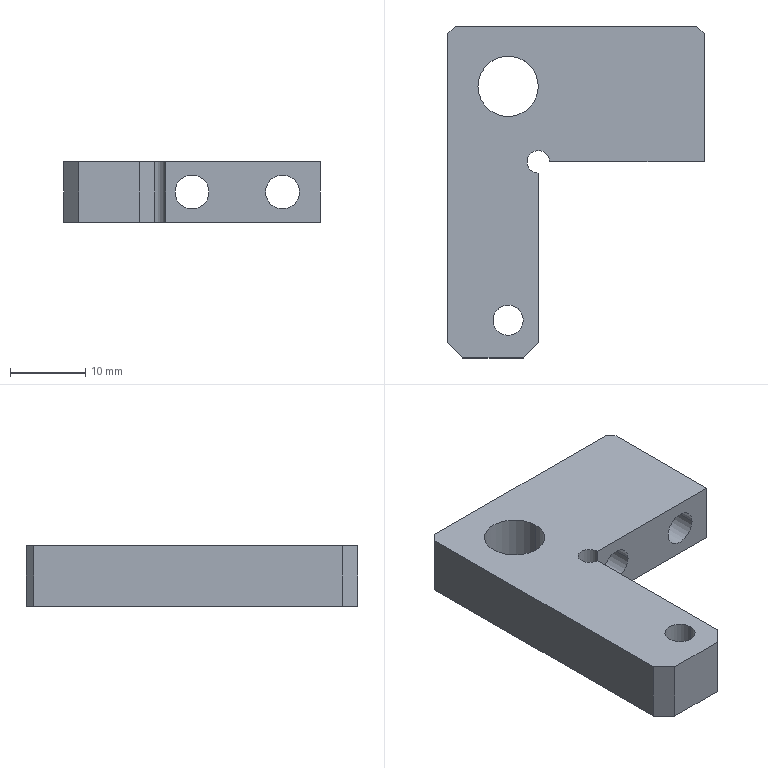Component | SolidWorks | A50-1 | 1 solid | 21 faces | box 34 x 44 x 8 mm | volume 6234 mm3 | plane 12 | cylinder 9 | commonest cylinder face diameters 4.5 x4 4 x2 8 x2 3 x1 | material S45C
build123d program:
from build123d import *

# Parameters (mm, degrees)
SKETCH1_W                  = 34
SKETCH1_H                  = 18
BOSS_EXTRUDE1_DEPTH        = 4
M8X1_0_TAPPED_HOLE1_D      = 8
CHAMFER1_SIZE              = 1
F_4_5_4_5_DIAMETER_HOLE1_D = 4.5
SKETCH11_W                 = 8
SKETCH11_H                 = 12
BOSS_EXTRUDE2_DEPTH        = 26
M4_TAPPED_HOLE2_D          = 4
CHAMFER3_SIZE              = 2
SKETCH14_R                 = 1.5
CUT_EXTRUDE2_DEPTH         = 40.724


with BuildPart() as part:
    # Sketch1 → Boss-Extrude1 (new, symmetric)
    with BuildSketch(Plane(origin=(0, 0, 0), x_dir=(0, 0, -1), z_dir=(1, 0, 0))):
        Rectangle(SKETCH1_W, SKETCH1_H)
    extrude(amount=BOSS_EXTRUDE1_DEPTH, both=True)

    # M8x1.0 Tapped Hole1 (through all)
    with Locations(Plane(origin=(4, 0, 0), x_dir=(0, 0, -1), z_dir=(1, 0, 0))):
        with Locations((9, -1)):
            Hole(M8X1_0_TAPPED_HOLE1_D / 2)

    # Chamfer1
    chamfer1_edges = [part.edges().sort_by_distance(p)[0] for p in [
        (0, -9, -17),
        (0, -9, 17),
    ]]
    chamfer(chamfer1_edges, length=CHAMFER1_SIZE)

    # 4.5 _4.5_ Diameter Hole1 (through all)
    with Locations(Plane(origin=(0, -9, 0), x_dir=(-1, 0, 0), z_dir=(0, -1, 0))):
        with Locations((0, -12), (0, 0)):
            Hole(F_4_5_4_5_DIAMETER_HOLE1_D / 2)

    # Sketch11 → Boss-Extrude2 (add)
    with BuildSketch(Plane(origin=(0, 9, 0), x_dir=(1, 0, 0), z_dir=(0, 1, 0))):
        with Locations((0, 11)):
            Rectangle(SKETCH11_W, SKETCH11_H)
    extrude(amount=BOSS_EXTRUDE2_DEPTH)

    # M4 Tapped Hole2 (through all)
    with Locations(Plane.ZY.offset(4)):
        with Locations((-9, 30)):
            Hole(M4_TAPPED_HOLE2_D / 2)

    # Chamfer3
    chamfer3_edges = [part.edges().sort_by_distance(p)[0] for p in [
        (0, 35, -5),
        (0, 35, -17),
    ]]
    chamfer(chamfer3_edges, length=CHAMFER3_SIZE)

    # Sketch14 → Cut-Extrude2 (cut, through all)
    with BuildSketch(Plane.ZY.offset(4)):
        with Locations((-5, 9)):
            Circle(SKETCH14_R)
    extrude(amount=-CUT_EXTRUDE2_DEPTH, mode=Mode.SUBTRACT)


solid = part.part

# Placed as in the assembly
solid = solid.moved(Location((-12.351, 41.364, -20), (180, 90, 0)))
STEP:
#1=CARTESIAN_POINT('',(-0.9193,0.4474,-0.6299));
#2=VERTEX_POINT('',#1);
#3=CARTESIAN_POINT('',(-0.7618,0.4474,-0.6299));
#4=VERTEX_POINT('',#3);
#5=CARTESIAN_POINT('',(-0.8406,0.4474,-0.6299));
#6=DIRECTION('',(0.,0.,-1.));
#7=DIRECTION('',(1.,0.,0.));
#8=AXIS2_PLACEMENT_3D('',#5,#6,#7);
#9=CIRCLE('',#8,0.07874);
#10=EDGE_CURVE('',#2,#4,#9,.T.);
#11=ORIENTED_EDGE('',*,*,#10,.F.);
#12=CARTESIAN_POINT('',(-0.9193,0.4474,-0.9449));
#13=VERTEX_POINT('',#12);
#14=CARTESIAN_POINT('',(-0.9193,0.4474,-0.9449));
#15=DIRECTION('',(0.,0.,-1.));
#16=VECTOR('',#15,39.37);
#17=LINE('',#14,#16);
#18=EDGE_CURVE('',#2,#13,#17,.T.);
#19=ORIENTED_EDGE('',*,*,#18,.T.);
#20=CARTESIAN_POINT('',(-0.7618,0.4474,-0.9449));
#21=VERTEX_POINT('',#20);
#22=CARTESIAN_POINT('',(-0.8406,0.4474,-0.9449));
#23=DIRECTION('',(0.,0.,-1.));
#24=DIRECTION('',(1.,0.,0.));
#25=AXIS2_PLACEMENT_3D('',#22,#23,#24);
#26=CIRCLE('',#25,0.07874);
#27=EDGE_CURVE('',#13,#21,#26,.T.);
#28=ORIENTED_EDGE('',*,*,#27,.T.);
#29=CARTESIAN_POINT('',(-0.7618,0.4474,-0.9449));
#30=DIRECTION('',(0.,0.,-1.));
#31=VECTOR('',#30,39.37);
#32=LINE('',#29,#31);
#33=EDGE_CURVE('',#4,#21,#32,.T.);
#34=ORIENTED_EDGE('',*,*,#33,.F.);
#35=EDGE_LOOP('',(#11,#19,#28,#34));
#36=FACE_OUTER_BOUND('',#35,.T.);
#37=CARTESIAN_POINT('',(-0.8406,0.4474,-0.9449));
#38=DIRECTION('',(0.,0.,-1.));
#39=DIRECTION('',(1.,0.,0.));
#40=AXIS2_PLACEMENT_3D('',#37,#38,#39);
#41=CYLINDRICAL_SURFACE('',#40,0.07874);
#42=ADVANCED_FACE('',(#36),#41,.F.);
#43=CARTESIAN_POINT('',(0.07477,1.274,-0.7874));
#44=VERTEX_POINT('',#43);
#45=CARTESIAN_POINT('',(-0.1024,1.274,-0.7874));
#46=VERTEX_POINT('',#45);
#47=CARTESIAN_POINT('',(-0.01381,1.274,-0.7874));
#48=DIRECTION('',(0.,1.,0.));
#49=DIRECTION('',(-1.,0.,0.));
#50=AXIS2_PLACEMENT_3D('',#47,#48,#49);
#51=CIRCLE('',#50,0.08858);
#52=EDGE_CURVE('',#44,#46,#51,.T.);
#53=ORIENTED_EDGE('',*,*,#52,.F.);
#54=CARTESIAN_POINT('',(0.07477,1.983,-0.7874));
#55=VERTEX_POINT('',#54);
#56=CARTESIAN_POINT('',(0.07477,1.983,-0.7874));
#57=DIRECTION('',(0.,1.,0.));
#58=VECTOR('',#57,39.37);
#59=LINE('',#56,#58);
#60=EDGE_CURVE('',#44,#55,#59,.T.);
#61=ORIENTED_EDGE('',*,*,#60,.T.);
#62=CARTESIAN_POINT('',(-0.1024,1.983,-0.7874));
#63=VERTEX_POINT('',#62);
#64=CARTESIAN_POINT('',(-0.01381,1.983,-0.7874));
#65=DIRECTION('',(0.,1.,0.));
#66=DIRECTION('',(-1.,0.,0.));
#67=AXIS2_PLACEMENT_3D('',#64,#65,#66);
#68=CIRCLE('',#67,0.08858);
#69=EDGE_CURVE('',#55,#63,#68,.T.);
#70=ORIENTED_EDGE('',*,*,#69,.T.);
#71=CARTESIAN_POINT('',(-0.1024,1.983,-0.7874));
#72=DIRECTION('',(0.,1.,0.));
#73=VECTOR('',#72,39.37);
#74=LINE('',#71,#73);
#75=EDGE_CURVE('',#46,#63,#74,.T.);
#76=ORIENTED_EDGE('',*,*,#75,.F.);
#77=EDGE_LOOP('',(#53,#61,#70,#76));
#78=FACE_OUTER_BOUND('',#77,.T.);
#79=CARTESIAN_POINT('',(-0.01381,1.983,-0.7874));
#80=DIRECTION('',(0.,1.,0.));
#81=DIRECTION('',(-1.,0.,0.));
#82=AXIS2_PLACEMENT_3D('',#79,#80,#81);
#83=CYLINDRICAL_SURFACE('',#82,0.08858);
#84=ADVANCED_FACE('',(#78),#83,.F.);
#85=CARTESIAN_POINT('',(-0.3977,1.274,-0.7874));
#86=VERTEX_POINT('',#85);
#87=CARTESIAN_POINT('',(-0.5748,1.274,-0.7874));
#88=VERTEX_POINT('',#87);
#89=CARTESIAN_POINT('',(-0.4863,1.274,-0.7874));
#90=DIRECTION('',(0.,1.,0.));
#91=DIRECTION('',(-1.,0.,0.));
#92=AXIS2_PLACEMENT_3D('',#89,#90,#91);
#93=CIRCLE('',#92,0.08858);
#94=EDGE_CURVE('',#86,#88,#93,.T.);
#95=ORIENTED_EDGE('',*,*,#94,.F.);
#96=CARTESIAN_POINT('',(-0.3977,1.983,-0.7874));
#97=VERTEX_POINT('',#96);
#98=CARTESIAN_POINT('',(-0.3977,1.983,-0.7874));
#99=DIRECTION('',(0.,1.,0.));
#100=VECTOR('',#99,39.37);
#101=LINE('',#98,#100);
#102=EDGE_CURVE('',#86,#97,#101,.T.);
#103=ORIENTED_EDGE('',*,*,#102,.T.);
#104=CARTESIAN_POINT('',(-0.5748,1.983,-0.7874));
#105=VERTEX_POINT('',#104);
#106=CARTESIAN_POINT('',(-0.4863,1.983,-0.7874));
#107=DIRECTION('',(0.,1.,0.));
#108=DIRECTION('',(-1.,0.,0.));
#109=AXIS2_PLACEMENT_3D('',#106,#107,#108);
#110=CIRCLE('',#109,0.08858);
#111=EDGE_CURVE('',#97,#105,#110,.T.);
#112=ORIENTED_EDGE('',*,*,#111,.T.);
#113=CARTESIAN_POINT('',(-0.5748,1.983,-0.7874));
#114=DIRECTION('',(0.,1.,0.));
#115=VECTOR('',#114,39.37);
#116=LINE('',#113,#115);
#117=EDGE_CURVE('',#88,#105,#116,.T.);
#118=ORIENTED_EDGE('',*,*,#117,.F.);
#119=EDGE_LOOP('',(#95,#103,#112,#118));
#120=FACE_OUTER_BOUND('',#119,.T.);
#121=CARTESIAN_POINT('',(-0.4863,1.983,-0.7874));
#122=DIRECTION('',(0.,1.,0.));
#123=DIRECTION('',(-1.,0.,0.));
#124=AXIS2_PLACEMENT_3D('',#121,#122,#123);
#125=CYLINDRICAL_SURFACE('',#124,0.08858);
#126=ADVANCED_FACE('',(#120),#125,.F.);
#127=CARTESIAN_POINT('',(-0.6831,1.668,-0.9449));
#128=VERTEX_POINT('',#127);
#129=CARTESIAN_POINT('',(-0.9981,1.668,-0.9449));
#130=VERTEX_POINT('',#129);
#131=CARTESIAN_POINT('',(-0.8406,1.668,-0.9449));
#132=DIRECTION('',(-0.,0.,1.));
#133=DIRECTION('',(-1.,0.,0.));
#134=AXIS2_PLACEMENT_3D('',#131,#132,#133);
#135=CIRCLE('',#134,0.1575);
#136=EDGE_CURVE('',#128,#130,#135,.T.);
#137=ORIENTED_EDGE('',*,*,#136,.F.);
#138=CARTESIAN_POINT('',(-0.6831,1.668,-0.6299));
#139=VERTEX_POINT('',#138);
#140=CARTESIAN_POINT('',(-0.6831,1.668,-0.6299));
#141=DIRECTION('',(-0.,0.,1.));
#142=VECTOR('',#141,39.37);
#143=LINE('',#140,#142);
#144=EDGE_CURVE('',#128,#139,#143,.T.);
#145=ORIENTED_EDGE('',*,*,#144,.T.);
#146=CARTESIAN_POINT('',(-0.9981,1.668,-0.6299));
#147=VERTEX_POINT('',#146);
#148=CARTESIAN_POINT('',(-0.8406,1.668,-0.6299));
#149=DIRECTION('',(-0.,0.,1.));
#150=DIRECTION('',(-1.,0.,0.));
#151=AXIS2_PLACEMENT_3D('',#148,#149,#150);
#152=CIRCLE('',#151,0.1575);
#153=EDGE_CURVE('',#139,#147,#152,.T.);
#154=ORIENTED_EDGE('',*,*,#153,.T.);
#155=CARTESIAN_POINT('',(-0.9981,1.668,-0.6299));
#156=DIRECTION('',(-0.,0.,1.));
#157=VECTOR('',#156,39.37);
#158=LINE('',#155,#157);
#159=EDGE_CURVE('',#130,#147,#158,.T.);
#160=ORIENTED_EDGE('',*,*,#159,.F.);
#161=EDGE_LOOP('',(#137,#145,#154,#160));
#162=FACE_OUTER_BOUND('',#161,.T.);
#163=CARTESIAN_POINT('',(-0.8406,1.668,-0.6299));
#164=DIRECTION('',(-0.,0.,1.));
#165=DIRECTION('',(-1.,0.,0.));
#166=AXIS2_PLACEMENT_3D('',#163,#164,#165);
#167=CYLINDRICAL_SURFACE('',#166,0.1575);
#168=ADVANCED_FACE('',(#162),#167,.F.);
#169=CARTESIAN_POINT('',(-0.4863,1.274,-0.7874));
#170=DIRECTION('',(0.,1.,0.));
#171=DIRECTION('',(-1.,0.,0.));
#172=AXIS2_PLACEMENT_3D('',#169,#170,#171);
#173=CIRCLE('',#172,0.08858);
#174=EDGE_CURVE('',#88,#86,#173,.T.);
#175=ORIENTED_EDGE('',*,*,#174,.T.);
#176=ORIENTED_EDGE('',*,*,#94,.T.);
#177=EDGE_LOOP('',(#175,#176));
#178=FACE_BOUND('',#177,.T.);
#179=CARTESIAN_POINT('',(-0.01381,1.274,-0.7874));
#180=DIRECTION('',(0.,1.,0.));
#181=DIRECTION('',(-1.,0.,0.));
#182=AXIS2_PLACEMENT_3D('',#179,#180,#181);
#183=CIRCLE('',#182,0.08858);
#184=EDGE_CURVE('',#46,#44,#183,.T.);
#185=ORIENTED_EDGE('',*,*,#184,.T.);
#186=ORIENTED_EDGE('',*,*,#52,.T.);
#187=EDGE_LOOP('',(#185,#186));
#188=FACE_BOUND('',#187,.T.);
#189=CARTESIAN_POINT('',(-0.624,1.274,-0.6299));
#190=VERTEX_POINT('',#189);
#191=CARTESIAN_POINT('',(0.183,1.274,-0.6299));
#192=VERTEX_POINT('',#191);
#193=CARTESIAN_POINT('',(0.183,1.274,-0.6299));
#194=DIRECTION('',(1.,-0.,-0.));
#195=VECTOR('',#194,39.37);
#196=LINE('',#193,#195);
#197=EDGE_CURVE('',#190,#192,#196,.T.);
#198=ORIENTED_EDGE('',*,*,#197,.F.);
#199=CARTESIAN_POINT('',(-0.624,1.274,-0.9449));
#200=VERTEX_POINT('',#199);
#201=CARTESIAN_POINT('',(-0.624,1.274,-0.6299));
#202=DIRECTION('',(0.,0.,-1.));
#203=VECTOR('',#202,39.37);
#204=LINE('',#201,#203);
#205=EDGE_CURVE('',#190,#200,#204,.T.);
#206=ORIENTED_EDGE('',*,*,#205,.T.);
#207=CARTESIAN_POINT('',(0.183,1.274,-0.9449));
#208=VERTEX_POINT('',#207);
#209=CARTESIAN_POINT('',(0.183,1.274,-0.9449));
#210=DIRECTION('',(1.,-0.,-0.));
#211=VECTOR('',#210,39.37);
#212=LINE('',#209,#211);
#213=EDGE_CURVE('',#200,#208,#212,.T.);
#214=ORIENTED_EDGE('',*,*,#213,.T.);
#215=CARTESIAN_POINT('',(0.183,1.274,-0.6299));
#216=DIRECTION('',(0.,0.,-1.));
#217=VECTOR('',#216,39.37);
#218=LINE('',#215,#217);
#219=EDGE_CURVE('',#192,#208,#218,.T.);
#220=ORIENTED_EDGE('',*,*,#219,.F.);
#221=EDGE_LOOP('',(#198,#206,#214,#220));
#222=FACE_OUTER_BOUND('',#221,.T.);
#223=CARTESIAN_POINT('',(0.183,1.274,-0.6299));
#224=DIRECTION('',(0.,1.,-0.));
#225=DIRECTION('',(-1.,0.,0.));
#226=AXIS2_PLACEMENT_3D('',#223,#224,#225);
#227=PLANE('',#226);
#228=ADVANCED_FACE('',(#178,#188,#222),#227,.F.);
#229=CARTESIAN_POINT('',(-0.4863,1.983,-0.7874));
#230=DIRECTION('',(0.,1.,0.));
#231=DIRECTION('',(-1.,0.,0.));
#232=AXIS2_PLACEMENT_3D('',#229,#230,#231);
#233=CIRCLE('',#232,0.08858);
#234=EDGE_CURVE('',#105,#97,#233,.T.);
#235=ORIENTED_EDGE('',*,*,#234,.F.);
#236=ORIENTED_EDGE('',*,*,#111,.F.);
#237=EDGE_LOOP('',(#235,#236));
#238=FACE_BOUND('',#237,.T.);
#239=CARTESIAN_POINT('',(0.1437,1.983,-0.6299));
#240=VERTEX_POINT('',#239);
#241=CARTESIAN_POINT('',(-1.116,1.983,-0.6299));
#242=VERTEX_POINT('',#241);
#243=CARTESIAN_POINT('',(0.183,1.983,-0.6299));
#244=DIRECTION('',(-1.,0.,0.));
#245=VECTOR('',#244,39.37);
#246=LINE('',#243,#245);
#247=EDGE_CURVE('',#240,#242,#246,.T.);
#248=ORIENTED_EDGE('',*,*,#247,.F.);
#249=CARTESIAN_POINT('',(0.1437,1.983,-0.9449));
#250=VERTEX_POINT('',#249);
#251=CARTESIAN_POINT('',(0.1437,1.983,-0.6299));
#252=DIRECTION('',(0.,0.,-1.));
#253=VECTOR('',#252,39.37);
#254=LINE('',#251,#253);
#255=EDGE_CURVE('',#240,#250,#254,.T.);
#256=ORIENTED_EDGE('',*,*,#255,.T.);
#257=CARTESIAN_POINT('',(-1.116,1.983,-0.9449));
#258=VERTEX_POINT('',#257);
#259=CARTESIAN_POINT('',(0.183,1.983,-0.9449));
#260=DIRECTION('',(-1.,0.,0.));
#261=VECTOR('',#260,39.37);
#262=LINE('',#259,#261);
#263=EDGE_CURVE('',#250,#258,#262,.T.);
#264=ORIENTED_EDGE('',*,*,#263,.T.);
#265=CARTESIAN_POINT('',(-1.116,1.983,-0.6299));
#266=DIRECTION('',(-0.,0.,1.));
#267=VECTOR('',#266,39.37);
#268=LINE('',#265,#267);
#269=EDGE_CURVE('',#258,#242,#268,.T.);
#270=ORIENTED_EDGE('',*,*,#269,.T.);
#271=EDGE_LOOP('',(#248,#256,#264,#270));
#272=FACE_OUTER_BOUND('',#271,.T.);
#273=CARTESIAN_POINT('',(-0.01381,1.983,-0.7874));
#274=DIRECTION('',(0.,1.,0.));
#275=DIRECTION('',(-1.,0.,0.));
#276=AXIS2_PLACEMENT_3D('',#273,#274,#275);
#277=CIRCLE('',#276,0.08858);
#278=EDGE_CURVE('',#63,#55,#277,.T.);
#279=ORIENTED_EDGE('',*,*,#278,.F.);
#280=ORIENTED_EDGE('',*,*,#69,.F.);
#281=EDGE_LOOP('',(#279,#280));
#282=FACE_BOUND('',#281,.T.);
#283=CARTESIAN_POINT('',(0.183,1.983,-0.6299));
#284=DIRECTION('',(-0.,-1.,0.));
#285=DIRECTION('',(1.,-0.,-0.));
#286=AXIS2_PLACEMENT_3D('',#283,#284,#285);
#287=PLANE('',#286);
#288=ADVANCED_FACE('',(#238,#272,#282),#287,.F.);
#289=CARTESIAN_POINT('',(-1.156,1.943,-0.9449));
#290=VERTEX_POINT('',#289);
#291=CARTESIAN_POINT('',(-1.156,0.3293,-0.9449));
#292=VERTEX_POINT('',#291);
#293=CARTESIAN_POINT('',(-1.156,1.274,-0.9449));
#294=DIRECTION('',(-0.,-1.,0.));
#295=VECTOR('',#294,39.37);
#296=LINE('',#293,#295);
#297=EDGE_CURVE('',#290,#292,#296,.T.);
#298=ORIENTED_EDGE('',*,*,#297,.T.);
#299=CARTESIAN_POINT('',(-1.156,0.3293,-0.6299));
#300=VERTEX_POINT('',#299);
#301=CARTESIAN_POINT('',(-1.156,0.3293,-0.6299));
#302=DIRECTION('',(-0.,0.,1.));
#303=VECTOR('',#302,39.37);
#304=LINE('',#301,#303);
#305=EDGE_CURVE('',#292,#300,#304,.T.);
#306=ORIENTED_EDGE('',*,*,#305,.T.);
#307=CARTESIAN_POINT('',(-1.156,1.943,-0.6299));
#308=VERTEX_POINT('',#307);
#309=CARTESIAN_POINT('',(-1.156,1.274,-0.6299));
#310=DIRECTION('',(-0.,-1.,0.));
#311=VECTOR('',#310,39.37);
#312=LINE('',#309,#311);
#313=EDGE_CURVE('',#308,#300,#312,.T.);
#314=ORIENTED_EDGE('',*,*,#313,.F.);
#315=CARTESIAN_POINT('',(-1.156,1.943,-0.6299));
#316=DIRECTION('',(0.,0.,-1.));
#317=VECTOR('',#316,39.37);
#318=LINE('',#315,#317);
#319=EDGE_CURVE('',#308,#290,#318,.T.);
#320=ORIENTED_EDGE('',*,*,#319,.T.);
#321=EDGE_LOOP('',(#298,#306,#314,#320));
#322=FACE_OUTER_BOUND('',#321,.T.);
#323=CARTESIAN_POINT('',(-1.156,1.274,-0.6299));
#324=DIRECTION('',(1.,-0.,0.));
#325=DIRECTION('',(-0.,0.,1.));
#326=AXIS2_PLACEMENT_3D('',#323,#324,#325);
#327=PLANE('',#326);
#328=ADVANCED_FACE('',(#322),#327,.F.);
#329=CARTESIAN_POINT('',(0.183,1.943,-0.9449));
#330=VERTEX_POINT('',#329);
#331=CARTESIAN_POINT('',(0.183,1.274,-0.9449));
#332=DIRECTION('',(-0.,1.,0.));
#333=VECTOR('',#332,39.37);
#334=LINE('',#331,#333);
#335=EDGE_CURVE('',#208,#330,#334,.T.);
#336=ORIENTED_EDGE('',*,*,#335,.T.);
#337=CARTESIAN_POINT('',(0.183,1.943,-0.6299));
#338=VERTEX_POINT('',#337);
#339=CARTESIAN_POINT('',(0.183,1.943,-0.6299));
#340=DIRECTION('',(-0.,0.,1.));
#341=VECTOR('',#340,39.37);
#342=LINE('',#339,#341);
#343=EDGE_CURVE('',#330,#338,#342,.T.);
#344=ORIENTED_EDGE('',*,*,#343,.T.);
#345=CARTESIAN_POINT('',(0.183,1.274,-0.6299));
#346=DIRECTION('',(-0.,1.,0.));
#347=VECTOR('',#346,39.37);
#348=LINE('',#345,#347);
#349=EDGE_CURVE('',#192,#338,#348,.T.);
#350=ORIENTED_EDGE('',*,*,#349,.F.);
#351=ORIENTED_EDGE('',*,*,#219,.T.);
#352=EDGE_LOOP('',(#336,#344,#350,#351));
#353=FACE_OUTER_BOUND('',#352,.T.);
#354=CARTESIAN_POINT('',(0.183,1.274,-0.6299));
#355=DIRECTION('',(-1.,-0.,0.));
#356=DIRECTION('',(0.,-1.,-0.));
#357=AXIS2_PLACEMENT_3D('',#354,#355,#356);
#358=PLANE('',#357);
#359=ADVANCED_FACE('',(#353),#358,.F.);
#360=CARTESIAN_POINT('',(-0.6831,1.215,-0.6299));
#361=VERTEX_POINT('',#360);
#362=CARTESIAN_POINT('',(-0.6831,1.274,-0.6299));
#363=DIRECTION('',(0.,0.,-1.));
#364=DIRECTION('',(1.,0.,0.));
#365=AXIS2_PLACEMENT_3D('',#362,#363,#364);
#366=CIRCLE('',#365,0.05906);
#367=EDGE_CURVE('',#361,#190,#366,.T.);
#368=ORIENTED_EDGE('',*,*,#367,.T.);
#369=ORIENTED_EDGE('',*,*,#197,.T.);
#370=ORIENTED_EDGE('',*,*,#349,.T.);
#371=CARTESIAN_POINT('',(0.005875,2.121,-0.6299));
#372=DIRECTION('',(-0.7071,0.7071,0.));
#373=VECTOR('',#372,39.37);
#374=LINE('',#371,#373);
#375=EDGE_CURVE('',#338,#240,#374,.T.);
#376=ORIENTED_EDGE('',*,*,#375,.T.);
#377=ORIENTED_EDGE('',*,*,#247,.T.);
#378=CARTESIAN_POINT('',(-0.9784,2.121,-0.6299));
#379=DIRECTION('',(-0.7071,-0.7071,0.));
#380=VECTOR('',#379,39.37);
#381=LINE('',#378,#380);
#382=EDGE_CURVE('',#242,#308,#381,.T.);
#383=ORIENTED_EDGE('',*,*,#382,.T.);
#384=ORIENTED_EDGE('',*,*,#313,.T.);
#385=CARTESIAN_POINT('',(-1.077,0.2506,-0.6299));
#386=VERTEX_POINT('',#385);
#387=CARTESIAN_POINT('',(-1.471,0.6443,-0.6299));
#388=DIRECTION('',(0.7071,-0.7071,-0.));
#389=VECTOR('',#388,39.37);
#390=LINE('',#387,#389);
#391=EDGE_CURVE('',#300,#386,#390,.T.);
#392=ORIENTED_EDGE('',*,*,#391,.T.);
#393=CARTESIAN_POINT('',(-0.7618,0.2506,-0.6299));
#394=VERTEX_POINT('',#393);
#395=CARTESIAN_POINT('',(-1.156,0.2506,-0.6299));
#396=DIRECTION('',(-1.,0.,0.));
#397=VECTOR('',#396,39.37);
#398=LINE('',#395,#397);
#399=EDGE_CURVE('',#394,#386,#398,.T.);
#400=ORIENTED_EDGE('',*,*,#399,.F.);
#401=CARTESIAN_POINT('',(-0.6831,0.3293,-0.6299));
#402=VERTEX_POINT('',#401);
#403=CARTESIAN_POINT('',(0.06493,1.077,-0.6299));
#404=DIRECTION('',(0.7071,0.7071,-0.));
#405=VECTOR('',#404,39.37);
#406=LINE('',#403,#405);
#407=EDGE_CURVE('',#394,#402,#406,.T.);
#408=ORIENTED_EDGE('',*,*,#407,.T.);
#409=CARTESIAN_POINT('',(-0.6831,0.2506,-0.6299));
#410=DIRECTION('',(0.,1.,0.));
#411=VECTOR('',#410,39.37);
#412=LINE('',#409,#411);
#413=EDGE_CURVE('',#402,#361,#412,.T.);
#414=ORIENTED_EDGE('',*,*,#413,.T.);
#415=EDGE_LOOP('',(#368,#369,#370,#376,#377,#383,#384,#392,#400,#408,#414));
#416=FACE_OUTER_BOUND('',#415,.T.);
#417=CARTESIAN_POINT('',(-0.8406,0.4474,-0.6299));
#418=DIRECTION('',(0.,0.,-1.));
#419=DIRECTION('',(1.,0.,0.));
#420=AXIS2_PLACEMENT_3D('',#417,#418,#419);
#421=CIRCLE('',#420,0.07874);
#422=EDGE_CURVE('',#4,#2,#421,.T.);
#423=ORIENTED_EDGE('',*,*,#422,.T.);
#424=ORIENTED_EDGE('',*,*,#10,.T.);
#425=EDGE_LOOP('',(#423,#424));
#426=FACE_BOUND('',#425,.T.);
#427=CARTESIAN_POINT('',(-0.8406,1.668,-0.6299));
#428=DIRECTION('',(-0.,0.,1.));
#429=DIRECTION('',(-1.,0.,0.));
#430=AXIS2_PLACEMENT_3D('',#427,#428,#429);
#431=CIRCLE('',#430,0.1575);
#432=EDGE_CURVE('',#147,#139,#431,.T.);
#433=ORIENTED_EDGE('',*,*,#432,.F.);
#434=ORIENTED_EDGE('',*,*,#153,.F.);
#435=EDGE_LOOP('',(#433,#434));
#436=FACE_BOUND('',#435,.T.);
#437=CARTESIAN_POINT('',(-0.4863,1.629,-0.6299));
#438=DIRECTION('',(0.,-0.,1.));
#439=DIRECTION('',(-1.,0.,0.));
#440=AXIS2_PLACEMENT_3D('',#437,#438,#439);
#441=PLANE('',#440);
#442=ADVANCED_FACE('',(#416,#426,#436),#441,.T.);
#443=CARTESIAN_POINT('',(-0.8406,0.4474,-0.9449));
#444=DIRECTION('',(0.,0.,-1.));
#445=DIRECTION('',(1.,0.,0.));
#446=AXIS2_PLACEMENT_3D('',#443,#444,#445);
#447=CIRCLE('',#446,0.07874);
#448=EDGE_CURVE('',#21,#13,#447,.T.);
#449=ORIENTED_EDGE('',*,*,#448,.F.);
#450=ORIENTED_EDGE('',*,*,#27,.F.);
#451=EDGE_LOOP('',(#449,#450));
#452=FACE_BOUND('',#451,.T.);
#453=CARTESIAN_POINT('',(-0.8406,1.668,-0.9449));
#454=DIRECTION('',(-0.,0.,1.));
#455=DIRECTION('',(-1.,0.,0.));
#456=AXIS2_PLACEMENT_3D('',#453,#454,#455);
#457=CIRCLE('',#456,0.1575);
#458=EDGE_CURVE('',#130,#128,#457,.T.);
#459=ORIENTED_EDGE('',*,*,#458,.T.);
#460=ORIENTED_EDGE('',*,*,#136,.T.);
#461=EDGE_LOOP('',(#459,#460));
#462=FACE_BOUND('',#461,.T.);
#463=ORIENTED_EDGE('',*,*,#213,.F.);
#464=CARTESIAN_POINT('',(-0.6831,1.215,-0.9449));
#465=VERTEX_POINT('',#464);
#466=CARTESIAN_POINT('',(-0.6831,1.274,-0.9449));
#467=DIRECTION('',(0.,0.,-1.));
#468=DIRECTION('',(1.,0.,0.));
#469=AXIS2_PLACEMENT_3D('',#466,#467,#468);
#470=CIRCLE('',#469,0.05906);
#471=EDGE_CURVE('',#465,#200,#470,.T.);
#472=ORIENTED_EDGE('',*,*,#471,.F.);
#473=CARTESIAN_POINT('',(-0.6831,0.3293,-0.9449));
#474=VERTEX_POINT('',#473);
#475=CARTESIAN_POINT('',(-0.6831,0.2506,-0.9449));
#476=DIRECTION('',(0.,1.,0.));
#477=VECTOR('',#476,39.37);
#478=LINE('',#475,#477);
#479=EDGE_CURVE('',#474,#465,#478,.T.);
#480=ORIENTED_EDGE('',*,*,#479,.F.);
#481=CARTESIAN_POINT('',(-0.7618,0.2506,-0.9449));
#482=VERTEX_POINT('',#481);
#483=CARTESIAN_POINT('',(-0.7618,0.2506,-0.9449));
#484=DIRECTION('',(-0.7071,-0.7071,0.));
#485=VECTOR('',#484,39.37);
#486=LINE('',#483,#485);
#487=EDGE_CURVE('',#474,#482,#486,.T.);
#488=ORIENTED_EDGE('',*,*,#487,.T.);
#489=CARTESIAN_POINT('',(-1.077,0.2506,-0.9449));
#490=VERTEX_POINT('',#489);
#491=CARTESIAN_POINT('',(-1.156,0.2506,-0.9449));
#492=DIRECTION('',(1.,-0.,0.));
#493=VECTOR('',#492,39.37);
#494=LINE('',#491,#493);
#495=EDGE_CURVE('',#490,#482,#494,.T.);
#496=ORIENTED_EDGE('',*,*,#495,.F.);
#497=CARTESIAN_POINT('',(-1.077,0.2506,-0.9449));
#498=DIRECTION('',(-0.7071,0.7071,0.));
#499=VECTOR('',#498,39.37);
#500=LINE('',#497,#499);
#501=EDGE_CURVE('',#490,#292,#500,.T.);
#502=ORIENTED_EDGE('',*,*,#501,.T.);
#503=ORIENTED_EDGE('',*,*,#297,.F.);
#504=CARTESIAN_POINT('',(-1.156,1.943,-0.9449));
#505=DIRECTION('',(0.7071,0.7071,-0.));
#506=VECTOR('',#505,39.37);
#507=LINE('',#504,#506);
#508=EDGE_CURVE('',#290,#258,#507,.T.);
#509=ORIENTED_EDGE('',*,*,#508,.T.);
#510=ORIENTED_EDGE('',*,*,#263,.F.);
#511=CARTESIAN_POINT('',(0.1437,1.983,-0.9449));
#512=DIRECTION('',(0.7071,-0.7071,-0.));
#513=VECTOR('',#512,39.37);
#514=LINE('',#511,#513);
#515=EDGE_CURVE('',#250,#330,#514,.T.);
#516=ORIENTED_EDGE('',*,*,#515,.T.);
#517=ORIENTED_EDGE('',*,*,#335,.F.);
#518=EDGE_LOOP('',(#463,#472,#480,#488,#496,#502,#503,#509,#510,#516,#517));
#519=FACE_OUTER_BOUND('',#518,.T.);
#520=CARTESIAN_POINT('',(-0.4863,1.629,-0.9449));
#521=DIRECTION('',(0.,-0.,1.));
#522=DIRECTION('',(-1.,0.,0.));
#523=AXIS2_PLACEMENT_3D('',#520,#521,#522);
#524=PLANE('',#523);
#525=ADVANCED_FACE('',(#452,#462,#519),#524,.F.);
#526=ORIENTED_EDGE('',*,*,#144,.F.);
#527=ORIENTED_EDGE('',*,*,#458,.F.);
#528=ORIENTED_EDGE('',*,*,#159,.T.);
#529=ORIENTED_EDGE('',*,*,#432,.T.);
#530=EDGE_LOOP('',(#526,#527,#528,#529));
#531=FACE_OUTER_BOUND('',#530,.T.);
#532=CARTESIAN_POINT('',(-0.8406,1.668,-0.6299));
#533=DIRECTION('',(-0.,0.,1.));
#534=DIRECTION('',(-1.,0.,0.));
#535=AXIS2_PLACEMENT_3D('',#532,#533,#534);
#536=CYLINDRICAL_SURFACE('',#535,0.1575);
#537=ADVANCED_FACE('',(#531),#536,.F.);
#538=ORIENTED_EDGE('',*,*,#375,.F.);
#539=ORIENTED_EDGE('',*,*,#343,.F.);
#540=ORIENTED_EDGE('',*,*,#515,.F.);
#541=ORIENTED_EDGE('',*,*,#255,.F.);
#542=EDGE_LOOP('',(#538,#539,#540,#541));
#543=FACE_OUTER_BOUND('',#542,.T.);
#544=CARTESIAN_POINT('',(0.1437,1.983,-0.6299));
#545=DIRECTION('',(-0.7071,-0.7071,-0.));
#546=DIRECTION('',(0.,0.,-1.));
#547=AXIS2_PLACEMENT_3D('',#544,#545,#546);
#548=PLANE('',#547);
#549=ADVANCED_FACE('',(#543),#548,.F.);
#550=ORIENTED_EDGE('',*,*,#382,.F.);
#551=ORIENTED_EDGE('',*,*,#269,.F.);
#552=ORIENTED_EDGE('',*,*,#508,.F.);
#553=ORIENTED_EDGE('',*,*,#319,.F.);
#554=EDGE_LOOP('',(#550,#551,#552,#553));
#555=FACE_OUTER_BOUND('',#554,.T.);
#556=CARTESIAN_POINT('',(-1.156,1.943,-0.6299));
#557=DIRECTION('',(0.7071,-0.7071,0.));
#558=DIRECTION('',(0.,0.,-1.));
#559=AXIS2_PLACEMENT_3D('',#556,#557,#558);
#560=PLANE('',#559);
#561=ADVANCED_FACE('',(#555),#560,.F.);
#562=ORIENTED_EDGE('',*,*,#102,.F.);
#563=ORIENTED_EDGE('',*,*,#174,.F.);
#564=ORIENTED_EDGE('',*,*,#117,.T.);
#565=ORIENTED_EDGE('',*,*,#234,.T.);
#566=EDGE_LOOP('',(#562,#563,#564,#565));
#567=FACE_OUTER_BOUND('',#566,.T.);
#568=CARTESIAN_POINT('',(-0.4863,1.983,-0.7874));
#569=DIRECTION('',(0.,1.,0.));
#570=DIRECTION('',(-1.,0.,0.));
#571=AXIS2_PLACEMENT_3D('',#568,#569,#570);
#572=CYLINDRICAL_SURFACE('',#571,0.08858);
#573=ADVANCED_FACE('',(#567),#572,.F.);
#574=ORIENTED_EDGE('',*,*,#60,.F.);
#575=ORIENTED_EDGE('',*,*,#184,.F.);
#576=ORIENTED_EDGE('',*,*,#75,.T.);
#577=ORIENTED_EDGE('',*,*,#278,.T.);
#578=EDGE_LOOP('',(#574,#575,#576,#577));
#579=FACE_OUTER_BOUND('',#578,.T.);
#580=CARTESIAN_POINT('',(-0.01381,1.983,-0.7874));
#581=DIRECTION('',(0.,1.,0.));
#582=DIRECTION('',(-1.,0.,0.));
#583=AXIS2_PLACEMENT_3D('',#580,#581,#582);
#584=CYLINDRICAL_SURFACE('',#583,0.08858);
#585=ADVANCED_FACE('',(#579),#584,.F.);
#586=ORIENTED_EDGE('',*,*,#479,.T.);
#587=CARTESIAN_POINT('',(-0.6831,1.215,-0.6299));
#588=DIRECTION('',(-0.,0.,1.));
#589=VECTOR('',#588,39.37);
#590=LINE('',#587,#589);
#591=EDGE_CURVE('',#465,#361,#590,.T.);
#592=ORIENTED_EDGE('',*,*,#591,.T.);
#593=ORIENTED_EDGE('',*,*,#413,.F.);
#594=CARTESIAN_POINT('',(-0.6831,0.3293,-0.9449));
#595=DIRECTION('',(0.,0.,-1.));
#596=VECTOR('',#595,39.37);
#597=LINE('',#594,#596);
#598=EDGE_CURVE('',#402,#474,#597,.T.);
#599=ORIENTED_EDGE('',*,*,#598,.T.);
#600=EDGE_LOOP('',(#586,#592,#593,#599));
#601=FACE_OUTER_BOUND('',#600,.T.);
#602=CARTESIAN_POINT('',(-0.6831,0.2506,-0.9449));
#603=DIRECTION('',(-1.,0.,-0.));
#604=DIRECTION('',(0.,0.,-1.));
#605=AXIS2_PLACEMENT_3D('',#602,#603,#604);
#606=PLANE('',#605);
#607=ADVANCED_FACE('',(#601),#606,.F.);
#608=ORIENTED_EDGE('',*,*,#399,.T.);
#609=CARTESIAN_POINT('',(-1.077,0.2506,-0.9449));
#610=DIRECTION('',(0.,0.,-1.));
#611=VECTOR('',#610,39.37);
#612=LINE('',#609,#611);
#613=EDGE_CURVE('',#386,#490,#612,.T.);
#614=ORIENTED_EDGE('',*,*,#613,.T.);
#615=ORIENTED_EDGE('',*,*,#495,.T.);
#616=CARTESIAN_POINT('',(-0.7618,0.2506,-0.6299));
#617=DIRECTION('',(-0.,0.,1.));
#618=VECTOR('',#617,39.37);
#619=LINE('',#616,#618);
#620=EDGE_CURVE('',#482,#394,#619,.T.);
#621=ORIENTED_EDGE('',*,*,#620,.T.);
#622=EDGE_LOOP('',(#608,#614,#615,#621));
#623=FACE_OUTER_BOUND('',#622,.T.);
#624=CARTESIAN_POINT('',(-0.4863,0.2506,-0.7874));
#625=DIRECTION('',(-0.,-1.,0.));
#626=DIRECTION('',(1.,-0.,-0.));
#627=AXIS2_PLACEMENT_3D('',#624,#625,#626);
#628=PLANE('',#627);
#629=ADVANCED_FACE('',(#623),#628,.T.);
#630=ORIENTED_EDGE('',*,*,#18,.F.);
#631=ORIENTED_EDGE('',*,*,#422,.F.);
#632=ORIENTED_EDGE('',*,*,#33,.T.);
#633=ORIENTED_EDGE('',*,*,#448,.T.);
#634=EDGE_LOOP('',(#630,#631,#632,#633));
#635=FACE_OUTER_BOUND('',#634,.T.);
#636=CARTESIAN_POINT('',(-0.8406,0.4474,-0.9449));
#637=DIRECTION('',(0.,0.,-1.));
#638=DIRECTION('',(1.,0.,0.));
#639=AXIS2_PLACEMENT_3D('',#636,#637,#638);
#640=CYLINDRICAL_SURFACE('',#639,0.07874);
#641=ADVANCED_FACE('',(#635),#640,.F.);
#642=ORIENTED_EDGE('',*,*,#391,.F.);
#643=ORIENTED_EDGE('',*,*,#305,.F.);
#644=ORIENTED_EDGE('',*,*,#501,.F.);
#645=ORIENTED_EDGE('',*,*,#613,.F.);
#646=EDGE_LOOP('',(#642,#643,#644,#645));
#647=FACE_OUTER_BOUND('',#646,.T.);
#648=CARTESIAN_POINT('',(-1.077,0.2506,-0.7874));
#649=DIRECTION('',(-0.7071,-0.7071,-0.));
#650=DIRECTION('',(-0.,0.,1.));
#651=AXIS2_PLACEMENT_3D('',#648,#649,#650);
#652=PLANE('',#651);
#653=ADVANCED_FACE('',(#647),#652,.T.);
#654=ORIENTED_EDGE('',*,*,#487,.F.);
#655=ORIENTED_EDGE('',*,*,#598,.F.);
#656=ORIENTED_EDGE('',*,*,#407,.F.);
#657=ORIENTED_EDGE('',*,*,#620,.F.);
#658=EDGE_LOOP('',(#654,#655,#656,#657));
#659=FACE_OUTER_BOUND('',#658,.T.);
#660=CARTESIAN_POINT('',(-0.7618,0.2506,-0.7874));
#661=DIRECTION('',(0.7071,-0.7071,0.));
#662=DIRECTION('',(0.,0.,-1.));
#663=AXIS2_PLACEMENT_3D('',#660,#661,#662);
#664=PLANE('',#663);
#665=ADVANCED_FACE('',(#659),#664,.T.);
#666=ORIENTED_EDGE('',*,*,#367,.F.);
#667=ORIENTED_EDGE('',*,*,#591,.F.);
#668=ORIENTED_EDGE('',*,*,#471,.T.);
#669=ORIENTED_EDGE('',*,*,#205,.F.);
#670=EDGE_LOOP('',(#666,#667,#668,#669));
#671=FACE_OUTER_BOUND('',#670,.T.);
#672=CARTESIAN_POINT('',(-0.6831,1.274,-0.6299));
#673=DIRECTION('',(0.,0.,-1.));
#674=DIRECTION('',(1.,0.,0.));
#675=AXIS2_PLACEMENT_3D('',#672,#673,#674);
#676=CYLINDRICAL_SURFACE('',#675,0.05906);
#677=ADVANCED_FACE('',(#671),#676,.F.);
#678=CLOSED_SHELL('',(#42,#84,#126,#168,#228,#288,#328,#359,#442,#525,#537,#549,#561,#573,#585,#607,#629,#641,#653,#665,#677));
#679=MANIFOLD_SOLID_BREP('',#678);
#680=CARTESIAN_POINT('',(0.,0.,0.));
#681=DIRECTION('',(0.,0.,1.));
#682=DIRECTION('',(1.,0.,0.));
#683=AXIS2_PLACEMENT_3D('',#680,#681,#682);
#684=(LENGTH_UNIT()NAMED_UNIT(*)SI_UNIT($,.METRE.));
#685=LENGTH_MEASURE_WITH_UNIT(LENGTH_MEASURE(0.0254),#684);
#686=DIMENSIONAL_EXPONENTS(1.,0.,0.,0.,0.,0.,0.);
#687=(CONVERSION_BASED_UNIT('',#685)LENGTH_UNIT()NAMED_UNIT(#686));
#688=UNCERTAINTY_MEASURE_WITH_UNIT(LENGTH_MEASURE(0.00001),#687,'','');
#689=(NAMED_UNIT(*)PLANE_ANGLE_UNIT()SI_UNIT($,.RADIAN.));
#690=(NAMED_UNIT(*)SI_UNIT($,.STERADIAN.)SOLID_ANGLE_UNIT());
#691=(GEOMETRIC_REPRESENTATION_CONTEXT(3)GLOBAL_UNCERTAINTY_ASSIGNED_CONTEXT((#688))GLOBAL_UNIT_ASSIGNED_CONTEXT((#687,#689,#690))REPRESENTATION_CONTEXT('',''));
#692=ADVANCED_BREP_SHAPE_REPRESENTATION('',(#679,#683),#691);
#693=COLOUR_RGB('',0.7922,0.8196,0.9333);
#694=FILL_AREA_STYLE_COLOUR('',#693);
#695=FILL_AREA_STYLE('',(#694));
#696=SURFACE_STYLE_FILL_AREA(#695);
#697=SURFACE_SIDE_STYLE('',(#696));
#698=SURFACE_STYLE_USAGE(.BOTH.,#697);
#699=PRESENTATION_STYLE_ASSIGNMENT((#698));
#700=STYLED_ITEM('',(#699),#679);
#701=(LENGTH_UNIT()NAMED_UNIT(*)SI_UNIT($,.METRE.));
#702=LENGTH_MEASURE_WITH_UNIT(LENGTH_MEASURE(0.0254),#701);
#703=DIMENSIONAL_EXPONENTS(1.,0.,0.,0.,0.,0.,0.);
#704=(CONVERSION_BASED_UNIT('',#702)LENGTH_UNIT()NAMED_UNIT(#703));
#705=UNCERTAINTY_MEASURE_WITH_UNIT(LENGTH_MEASURE(0.00001),#704,'','');
#706=(NAMED_UNIT(*)PLANE_ANGLE_UNIT()SI_UNIT($,.RADIAN.));
#707=(NAMED_UNIT(*)SI_UNIT($,.STERADIAN.)SOLID_ANGLE_UNIT());
#708=(GEOMETRIC_REPRESENTATION_CONTEXT(3)GLOBAL_UNCERTAINTY_ASSIGNED_CONTEXT((#705))GLOBAL_UNIT_ASSIGNED_CONTEXT((#704,#706,#707))REPRESENTATION_CONTEXT('',''));
#709=MECHANICAL_DESIGN_GEOMETRIC_PRESENTATION_REPRESENTATION('',(#700),#708);
#710=PRESENTATION_LAYER_ASSIGNMENT('','',(#700));